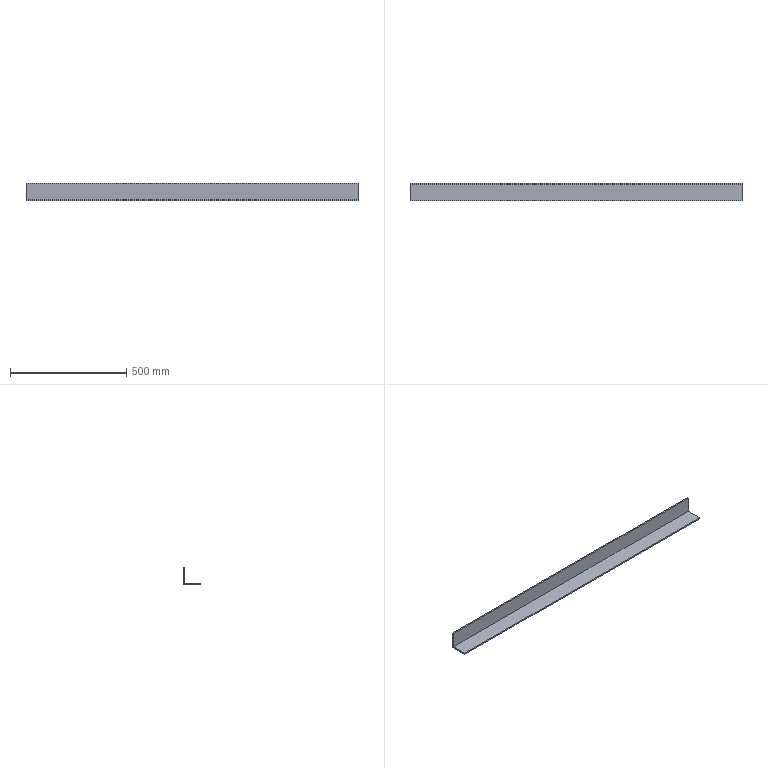Component | NX | DOWN_FRAME1430_2 | 1 solid | 8 faces | box 1430 x 75 x 75 mm | volume 1235520 mm3 | plane 8
STEP:
#1=CARTESIAN_POINT('',(0.,0.,0.));
#2=DIRECTION('',(0.,0.,1.));
#3=DIRECTION('',(1.,0.,0.));
#4=AXIS2_PLACEMENT_3D('',#1,#2,#3);
#5=CARTESIAN_POINT('',(0.,-6.,75.));
#6=VERTEX_POINT('',#5);
#7=CARTESIAN_POINT('',(0.,-6.,6.));
#8=VERTEX_POINT('',#7);
#9=CARTESIAN_POINT('',(0.,-6.,75.));
#10=DIRECTION('',(0.,0.,-1.));
#11=VECTOR('',#10,1.);
#12=LINE('',#9,#11);
#13=CARTESIAN_POINT('',(1430.,-6.,75.));
#14=DIRECTION('',(0.,1.,0.));
#15=DIRECTION('',(-1.,0.,0.));
#16=AXIS2_PLACEMENT_3D('',#13,#14,#15);
#17=PLANE('',#16);
#18=CARTESIAN_POINT('',(1430.,0.));
#19=DIRECTION('',(0.,-1.));
#20=VECTOR('',#19,1.);
#21=LINE('',#18,#20);
#22=(GEOMETRIC_REPRESENTATION_CONTEXT(2)PARAMETRIC_REPRESENTATION_CONTEXT()REPRESENTATION_CONTEXT('',''));
#23=DEFINITIONAL_REPRESENTATION('',(#21),#22);
#24=PCURVE('',#17,#23);
#25=CARTESIAN_POINT('',(0.,-6.,6.));
#26=DIRECTION('',(-1.,0.,0.));
#27=DIRECTION('',(0.,-1.,0.));
#28=AXIS2_PLACEMENT_3D('',#25,#26,#27);
#29=PLANE('',#28);
#30=CARTESIAN_POINT('',(0.,69.));
#31=DIRECTION('',(0.,-1.));
#32=VECTOR('',#31,1.);
#33=LINE('',#30,#32);
#34=(GEOMETRIC_REPRESENTATION_CONTEXT(2)PARAMETRIC_REPRESENTATION_CONTEXT()REPRESENTATION_CONTEXT('',''));
#35=DEFINITIONAL_REPRESENTATION('',(#33),#34);
#36=PCURVE('',#29,#35);
#37=SURFACE_CURVE('',#12,(#24,#36),.PCURVE_S1.);
#38=EDGE_CURVE('',#6,#8,#37,.T.);
#39=ORIENTED_EDGE('',*,*,#38,.T.);
#40=CARTESIAN_POINT('',(1430.,-6.,6.));
#41=VERTEX_POINT('',#40);
#42=CARTESIAN_POINT('',(1430.,-6.,6.));
#43=DIRECTION('',(-1.,0.,0.));
#44=VECTOR('',#43,1.);
#45=LINE('',#42,#44);
#46=CARTESIAN_POINT('',(0.,-69.));
#47=DIRECTION('',(1.,0.));
#48=VECTOR('',#47,1.);
#49=LINE('',#46,#48);
#50=(GEOMETRIC_REPRESENTATION_CONTEXT(2)PARAMETRIC_REPRESENTATION_CONTEXT()REPRESENTATION_CONTEXT('',''));
#51=DEFINITIONAL_REPRESENTATION('',(#49),#50);
#52=PCURVE('',#17,#51);
#53=CARTESIAN_POINT('',(1430.,-6.,6.));
#54=DIRECTION('',(0.,-0.,-1.));
#55=DIRECTION('',(0.,1.,-0.));
#56=AXIS2_PLACEMENT_3D('',#53,#54,#55);
#57=PLANE('',#56);
#58=CARTESIAN_POINT('',(0.,0.));
#59=DIRECTION('',(0.,-1.));
#60=VECTOR('',#59,1.);
#61=LINE('',#58,#60);
#62=(GEOMETRIC_REPRESENTATION_CONTEXT(2)PARAMETRIC_REPRESENTATION_CONTEXT()REPRESENTATION_CONTEXT('',''));
#63=DEFINITIONAL_REPRESENTATION('',(#61),#62);
#64=PCURVE('',#57,#63);
#65=SURFACE_CURVE('',#45,(#52,#64),.PCURVE_S1.);
#66=EDGE_CURVE('',#41,#8,#65,.T.);
#67=ORIENTED_EDGE('',*,*,#66,.F.);
#68=CARTESIAN_POINT('',(1430.,-6.,75.));
#69=VERTEX_POINT('',#68);
#70=CARTESIAN_POINT('',(1430.,-6.,75.));
#71=DIRECTION('',(0.,0.,-1.));
#72=VECTOR('',#71,1.);
#73=LINE('',#70,#72);
#74=CARTESIAN_POINT('',(0.,0.));
#75=DIRECTION('',(0.,-1.));
#76=VECTOR('',#75,1.);
#77=LINE('',#74,#76);
#78=(GEOMETRIC_REPRESENTATION_CONTEXT(2)PARAMETRIC_REPRESENTATION_CONTEXT()REPRESENTATION_CONTEXT('',''));
#79=DEFINITIONAL_REPRESENTATION('',(#77),#78);
#80=PCURVE('',#17,#79);
#81=CARTESIAN_POINT('',(1430.,-6.,6.));
#82=DIRECTION('',(-1.,0.,0.));
#83=DIRECTION('',(0.,-1.,0.));
#84=AXIS2_PLACEMENT_3D('',#81,#82,#83);
#85=PLANE('',#84);
#86=CARTESIAN_POINT('',(0.,69.));
#87=DIRECTION('',(0.,-1.));
#88=VECTOR('',#87,1.);
#89=LINE('',#86,#88);
#90=(GEOMETRIC_REPRESENTATION_CONTEXT(2)PARAMETRIC_REPRESENTATION_CONTEXT()REPRESENTATION_CONTEXT('',''));
#91=DEFINITIONAL_REPRESENTATION('',(#89),#90);
#92=PCURVE('',#85,#91);
#93=SURFACE_CURVE('',#73,(#80,#92),.PCURVE_S1.);
#94=EDGE_CURVE('',#69,#41,#93,.T.);
#95=ORIENTED_EDGE('',*,*,#94,.F.);
#96=CARTESIAN_POINT('',(1430.,-6.,75.));
#97=DIRECTION('',(-1.,0.,0.));
#98=VECTOR('',#97,1.);
#99=LINE('',#96,#98);
#100=CARTESIAN_POINT('',(0.,0.));
#101=DIRECTION('',(1.,0.));
#102=VECTOR('',#101,1.);
#103=LINE('',#100,#102);
#104=(GEOMETRIC_REPRESENTATION_CONTEXT(2)PARAMETRIC_REPRESENTATION_CONTEXT()REPRESENTATION_CONTEXT('',''));
#105=DEFINITIONAL_REPRESENTATION('',(#103),#104);
#106=PCURVE('',#17,#105);
#107=CARTESIAN_POINT('',(1430.,0.,75.));
#108=DIRECTION('',(0.,0.,-1.));
#109=DIRECTION('',(0.,1.,0.));
#110=AXIS2_PLACEMENT_3D('',#107,#108,#109);
#111=PLANE('',#110);
#112=CARTESIAN_POINT('',(-6.,0.));
#113=DIRECTION('',(0.,-1.));
#114=VECTOR('',#113,1.);
#115=LINE('',#112,#114);
#116=(GEOMETRIC_REPRESENTATION_CONTEXT(2)PARAMETRIC_REPRESENTATION_CONTEXT()REPRESENTATION_CONTEXT('',''));
#117=DEFINITIONAL_REPRESENTATION('',(#115),#116);
#118=PCURVE('',#111,#117);
#119=SURFACE_CURVE('',#99,(#106,#118),.PCURVE_S1.);
#120=EDGE_CURVE('',#69,#6,#119,.T.);
#121=ORIENTED_EDGE('',*,*,#120,.T.);
#122=EDGE_LOOP('',(#39,#67,#95,#121));
#123=FACE_BOUND('',#122,.T.);
#124=ADVANCED_FACE('',(#123),#17,.F.);
#125=CARTESIAN_POINT('',(0.,-75.,6.));
#126=VERTEX_POINT('',#125);
#127=CARTESIAN_POINT('',(0.,-6.,6.));
#128=DIRECTION('',(0.,-1.,0.));
#129=VECTOR('',#128,1.);
#130=LINE('',#127,#129);
#131=CARTESIAN_POINT('',(0.,-1430.));
#132=DIRECTION('',(-1.,0.));
#133=VECTOR('',#132,1.);
#134=LINE('',#131,#133);
#135=(GEOMETRIC_REPRESENTATION_CONTEXT(2)PARAMETRIC_REPRESENTATION_CONTEXT()REPRESENTATION_CONTEXT('',''));
#136=DEFINITIONAL_REPRESENTATION('',(#134),#135);
#137=PCURVE('',#57,#136);
#138=CARTESIAN_POINT('',(0.,0.));
#139=DIRECTION('',(1.,0.));
#140=VECTOR('',#139,1.);
#141=LINE('',#138,#140);
#142=(GEOMETRIC_REPRESENTATION_CONTEXT(2)PARAMETRIC_REPRESENTATION_CONTEXT()REPRESENTATION_CONTEXT('',''));
#143=DEFINITIONAL_REPRESENTATION('',(#141),#142);
#144=PCURVE('',#29,#143);
#145=SURFACE_CURVE('',#130,(#137,#144),.PCURVE_S1.);
#146=EDGE_CURVE('',#8,#126,#145,.T.);
#147=ORIENTED_EDGE('',*,*,#146,.T.);
#148=CARTESIAN_POINT('',(1430.,-75.,6.));
#149=VERTEX_POINT('',#148);
#150=CARTESIAN_POINT('',(1430.,-75.,6.));
#151=DIRECTION('',(-1.,0.,0.));
#152=VECTOR('',#151,1.);
#153=LINE('',#150,#152);
#154=CARTESIAN_POINT('',(-69.,0.));
#155=DIRECTION('',(0.,-1.));
#156=VECTOR('',#155,1.);
#157=LINE('',#154,#156);
#158=(GEOMETRIC_REPRESENTATION_CONTEXT(2)PARAMETRIC_REPRESENTATION_CONTEXT()REPRESENTATION_CONTEXT('',''));
#159=DEFINITIONAL_REPRESENTATION('',(#157),#158);
#160=PCURVE('',#57,#159);
#161=CARTESIAN_POINT('',(1430.,-75.,6.));
#162=DIRECTION('',(0.,1.,0.));
#163=DIRECTION('',(-1.,0.,0.));
#164=AXIS2_PLACEMENT_3D('',#161,#162,#163);
#165=PLANE('',#164);
#166=CARTESIAN_POINT('',(0.,0.));
#167=DIRECTION('',(1.,0.));
#168=VECTOR('',#167,1.);
#169=LINE('',#166,#168);
#170=(GEOMETRIC_REPRESENTATION_CONTEXT(2)PARAMETRIC_REPRESENTATION_CONTEXT()REPRESENTATION_CONTEXT('',''));
#171=DEFINITIONAL_REPRESENTATION('',(#169),#170);
#172=PCURVE('',#165,#171);
#173=SURFACE_CURVE('',#153,(#160,#172),.PCURVE_S1.);
#174=EDGE_CURVE('',#149,#126,#173,.T.);
#175=ORIENTED_EDGE('',*,*,#174,.F.);
#176=CARTESIAN_POINT('',(1430.,-6.,6.));
#177=DIRECTION('',(0.,-1.,0.));
#178=VECTOR('',#177,1.);
#179=LINE('',#176,#178);
#180=CARTESIAN_POINT('',(0.,0.));
#181=DIRECTION('',(-1.,0.));
#182=VECTOR('',#181,1.);
#183=LINE('',#180,#182);
#184=(GEOMETRIC_REPRESENTATION_CONTEXT(2)PARAMETRIC_REPRESENTATION_CONTEXT()REPRESENTATION_CONTEXT('',''));
#185=DEFINITIONAL_REPRESENTATION('',(#183),#184);
#186=PCURVE('',#57,#185);
#187=CARTESIAN_POINT('',(0.,0.));
#188=DIRECTION('',(1.,0.));
#189=VECTOR('',#188,1.);
#190=LINE('',#187,#189);
#191=(GEOMETRIC_REPRESENTATION_CONTEXT(2)PARAMETRIC_REPRESENTATION_CONTEXT()REPRESENTATION_CONTEXT('',''));
#192=DEFINITIONAL_REPRESENTATION('',(#190),#191);
#193=PCURVE('',#85,#192);
#194=SURFACE_CURVE('',#179,(#186,#193),.PCURVE_S1.);
#195=EDGE_CURVE('',#41,#149,#194,.T.);
#196=ORIENTED_EDGE('',*,*,#195,.F.);
#197=ORIENTED_EDGE('',*,*,#66,.T.);
#198=EDGE_LOOP('',(#147,#175,#196,#197));
#199=FACE_BOUND('',#198,.T.);
#200=ADVANCED_FACE('',(#199),#57,.F.);
#201=CARTESIAN_POINT('',(0.,-75.,0.));
#202=VERTEX_POINT('',#201);
#203=CARTESIAN_POINT('',(0.,-75.,6.));
#204=DIRECTION('',(0.,0.,-1.));
#205=VECTOR('',#204,1.);
#206=LINE('',#203,#205);
#207=CARTESIAN_POINT('',(1430.,0.));
#208=DIRECTION('',(0.,-1.));
#209=VECTOR('',#208,1.);
#210=LINE('',#207,#209);
#211=(GEOMETRIC_REPRESENTATION_CONTEXT(2)PARAMETRIC_REPRESENTATION_CONTEXT()REPRESENTATION_CONTEXT('',''));
#212=DEFINITIONAL_REPRESENTATION('',(#210),#211);
#213=PCURVE('',#165,#212);
#214=CARTESIAN_POINT('',(69.,0.));
#215=DIRECTION('',(0.,-1.));
#216=VECTOR('',#215,1.);
#217=LINE('',#214,#216);
#218=(GEOMETRIC_REPRESENTATION_CONTEXT(2)PARAMETRIC_REPRESENTATION_CONTEXT()REPRESENTATION_CONTEXT('',''));
#219=DEFINITIONAL_REPRESENTATION('',(#217),#218);
#220=PCURVE('',#29,#219);
#221=SURFACE_CURVE('',#206,(#213,#220),.PCURVE_S1.);
#222=EDGE_CURVE('',#126,#202,#221,.T.);
#223=ORIENTED_EDGE('',*,*,#222,.T.);
#224=CARTESIAN_POINT('',(1430.,-75.,0.));
#225=VERTEX_POINT('',#224);
#226=CARTESIAN_POINT('',(1430.,-75.,0.));
#227=DIRECTION('',(-1.,0.,0.));
#228=VECTOR('',#227,1.);
#229=LINE('',#226,#228);
#230=CARTESIAN_POINT('',(0.,-6.));
#231=DIRECTION('',(1.,0.));
#232=VECTOR('',#231,1.);
#233=LINE('',#230,#232);
#234=(GEOMETRIC_REPRESENTATION_CONTEXT(2)PARAMETRIC_REPRESENTATION_CONTEXT()REPRESENTATION_CONTEXT('',''));
#235=DEFINITIONAL_REPRESENTATION('',(#233),#234);
#236=PCURVE('',#165,#235);
#237=CARTESIAN_POINT('',(1430.,-75.,0.));
#238=DIRECTION('',(0.,0.,1.));
#239=DIRECTION('',(0.,-1.,0.));
#240=AXIS2_PLACEMENT_3D('',#237,#238,#239);
#241=PLANE('',#240);
#242=CARTESIAN_POINT('',(0.,0.));
#243=DIRECTION('',(0.,-1.));
#244=VECTOR('',#243,1.);
#245=LINE('',#242,#244);
#246=(GEOMETRIC_REPRESENTATION_CONTEXT(2)PARAMETRIC_REPRESENTATION_CONTEXT()REPRESENTATION_CONTEXT('',''));
#247=DEFINITIONAL_REPRESENTATION('',(#245),#246);
#248=PCURVE('',#241,#247);
#249=SURFACE_CURVE('',#229,(#236,#248),.PCURVE_S1.);
#250=EDGE_CURVE('',#225,#202,#249,.T.);
#251=ORIENTED_EDGE('',*,*,#250,.F.);
#252=CARTESIAN_POINT('',(1430.,-75.,6.));
#253=DIRECTION('',(0.,0.,-1.));
#254=VECTOR('',#253,1.);
#255=LINE('',#252,#254);
#256=CARTESIAN_POINT('',(0.,0.));
#257=DIRECTION('',(0.,-1.));
#258=VECTOR('',#257,1.);
#259=LINE('',#256,#258);
#260=(GEOMETRIC_REPRESENTATION_CONTEXT(2)PARAMETRIC_REPRESENTATION_CONTEXT()REPRESENTATION_CONTEXT('',''));
#261=DEFINITIONAL_REPRESENTATION('',(#259),#260);
#262=PCURVE('',#165,#261);
#263=CARTESIAN_POINT('',(69.,0.));
#264=DIRECTION('',(0.,-1.));
#265=VECTOR('',#264,1.);
#266=LINE('',#263,#265);
#267=(GEOMETRIC_REPRESENTATION_CONTEXT(2)PARAMETRIC_REPRESENTATION_CONTEXT()REPRESENTATION_CONTEXT('',''));
#268=DEFINITIONAL_REPRESENTATION('',(#266),#267);
#269=PCURVE('',#85,#268);
#270=SURFACE_CURVE('',#255,(#262,#269),.PCURVE_S1.);
#271=EDGE_CURVE('',#149,#225,#270,.T.);
#272=ORIENTED_EDGE('',*,*,#271,.F.);
#273=ORIENTED_EDGE('',*,*,#174,.T.);
#274=EDGE_LOOP('',(#223,#251,#272,#273));
#275=FACE_BOUND('',#274,.T.);
#276=ADVANCED_FACE('',(#275),#165,.F.);
#277=CARTESIAN_POINT('',(0.,0.,0.));
#278=VERTEX_POINT('',#277);
#279=CARTESIAN_POINT('',(0.,-75.,0.));
#280=DIRECTION('',(0.,1.,-0.));
#281=VECTOR('',#280,1.);
#282=LINE('',#279,#281);
#283=CARTESIAN_POINT('',(0.,-1430.));
#284=DIRECTION('',(-1.,0.));
#285=VECTOR('',#284,1.);
#286=LINE('',#283,#285);
#287=(GEOMETRIC_REPRESENTATION_CONTEXT(2)PARAMETRIC_REPRESENTATION_CONTEXT()REPRESENTATION_CONTEXT('',''));
#288=DEFINITIONAL_REPRESENTATION('',(#286),#287);
#289=PCURVE('',#241,#288);
#290=CARTESIAN_POINT('',(69.,-6.));
#291=DIRECTION('',(-1.,-0.));
#292=VECTOR('',#291,1.);
#293=LINE('',#290,#292);
#294=(GEOMETRIC_REPRESENTATION_CONTEXT(2)PARAMETRIC_REPRESENTATION_CONTEXT()REPRESENTATION_CONTEXT('',''));
#295=DEFINITIONAL_REPRESENTATION('',(#293),#294);
#296=PCURVE('',#29,#295);
#297=SURFACE_CURVE('',#282,(#289,#296),.PCURVE_S1.);
#298=EDGE_CURVE('',#202,#278,#297,.T.);
#299=ORIENTED_EDGE('',*,*,#298,.T.);
#300=CARTESIAN_POINT('',(1430.,0.,0.));
#301=VERTEX_POINT('',#300);
#302=CARTESIAN_POINT('',(1430.,0.,0.));
#303=DIRECTION('',(-1.,0.,0.));
#304=VECTOR('',#303,1.);
#305=LINE('',#302,#304);
#306=CARTESIAN_POINT('',(-75.,0.));
#307=DIRECTION('',(0.,-1.));
#308=VECTOR('',#307,1.);
#309=LINE('',#306,#308);
#310=(GEOMETRIC_REPRESENTATION_CONTEXT(2)PARAMETRIC_REPRESENTATION_CONTEXT()REPRESENTATION_CONTEXT('',''));
#311=DEFINITIONAL_REPRESENTATION('',(#309),#310);
#312=PCURVE('',#241,#311);
#313=CARTESIAN_POINT('',(1430.,0.,0.));
#314=DIRECTION('',(0.,-1.,0.));
#315=DIRECTION('',(1.,0.,0.));
#316=AXIS2_PLACEMENT_3D('',#313,#314,#315);
#317=PLANE('',#316);
#318=CARTESIAN_POINT('',(0.,0.));
#319=DIRECTION('',(-1.,0.));
#320=VECTOR('',#319,1.);
#321=LINE('',#318,#320);
#322=(GEOMETRIC_REPRESENTATION_CONTEXT(2)PARAMETRIC_REPRESENTATION_CONTEXT()REPRESENTATION_CONTEXT('',''));
#323=DEFINITIONAL_REPRESENTATION('',(#321),#322);
#324=PCURVE('',#317,#323);
#325=SURFACE_CURVE('',#305,(#312,#324),.PCURVE_S1.);
#326=EDGE_CURVE('',#301,#278,#325,.T.);
#327=ORIENTED_EDGE('',*,*,#326,.F.);
#328=CARTESIAN_POINT('',(1430.,-75.,0.));
#329=DIRECTION('',(0.,1.,-0.));
#330=VECTOR('',#329,1.);
#331=LINE('',#328,#330);
#332=CARTESIAN_POINT('',(0.,0.));
#333=DIRECTION('',(-1.,0.));
#334=VECTOR('',#333,1.);
#335=LINE('',#332,#334);
#336=(GEOMETRIC_REPRESENTATION_CONTEXT(2)PARAMETRIC_REPRESENTATION_CONTEXT()REPRESENTATION_CONTEXT('',''));
#337=DEFINITIONAL_REPRESENTATION('',(#335),#336);
#338=PCURVE('',#241,#337);
#339=CARTESIAN_POINT('',(69.,-6.));
#340=DIRECTION('',(-1.,-0.));
#341=VECTOR('',#340,1.);
#342=LINE('',#339,#341);
#343=(GEOMETRIC_REPRESENTATION_CONTEXT(2)PARAMETRIC_REPRESENTATION_CONTEXT()REPRESENTATION_CONTEXT('',''));
#344=DEFINITIONAL_REPRESENTATION('',(#342),#343);
#345=PCURVE('',#85,#344);
#346=SURFACE_CURVE('',#331,(#338,#345),.PCURVE_S1.);
#347=EDGE_CURVE('',#225,#301,#346,.T.);
#348=ORIENTED_EDGE('',*,*,#347,.F.);
#349=ORIENTED_EDGE('',*,*,#250,.T.);
#350=EDGE_LOOP('',(#299,#327,#348,#349));
#351=FACE_BOUND('',#350,.T.);
#352=ADVANCED_FACE('',(#351),#241,.F.);
#353=CARTESIAN_POINT('',(0.,0.,75.));
#354=VERTEX_POINT('',#353);
#355=CARTESIAN_POINT('',(0.,0.,0.));
#356=DIRECTION('',(0.,0.,1.));
#357=VECTOR('',#356,1.);
#358=LINE('',#355,#357);
#359=CARTESIAN_POINT('',(-1430.,0.));
#360=DIRECTION('',(0.,1.));
#361=VECTOR('',#360,1.);
#362=LINE('',#359,#361);
#363=(GEOMETRIC_REPRESENTATION_CONTEXT(2)PARAMETRIC_REPRESENTATION_CONTEXT()REPRESENTATION_CONTEXT('',''));
#364=DEFINITIONAL_REPRESENTATION('',(#362),#363);
#365=PCURVE('',#317,#364);
#366=CARTESIAN_POINT('',(-6.,-6.));
#367=DIRECTION('',(0.,1.));
#368=VECTOR('',#367,1.);
#369=LINE('',#366,#368);
#370=(GEOMETRIC_REPRESENTATION_CONTEXT(2)PARAMETRIC_REPRESENTATION_CONTEXT()REPRESENTATION_CONTEXT('',''));
#371=DEFINITIONAL_REPRESENTATION('',(#369),#370);
#372=PCURVE('',#29,#371);
#373=SURFACE_CURVE('',#358,(#365,#372),.PCURVE_S1.);
#374=EDGE_CURVE('',#278,#354,#373,.T.);
#375=ORIENTED_EDGE('',*,*,#374,.T.);
#376=CARTESIAN_POINT('',(1430.,0.,75.));
#377=VERTEX_POINT('',#376);
#378=CARTESIAN_POINT('',(1430.,0.,75.));
#379=DIRECTION('',(-1.,0.,0.));
#380=VECTOR('',#379,1.);
#381=LINE('',#378,#380);
#382=CARTESIAN_POINT('',(0.,75.));
#383=DIRECTION('',(-1.,0.));
#384=VECTOR('',#383,1.);
#385=LINE('',#382,#384);
#386=(GEOMETRIC_REPRESENTATION_CONTEXT(2)PARAMETRIC_REPRESENTATION_CONTEXT()REPRESENTATION_CONTEXT('',''));
#387=DEFINITIONAL_REPRESENTATION('',(#385),#386);
#388=PCURVE('',#317,#387);
#389=CARTESIAN_POINT('',(0.,0.));
#390=DIRECTION('',(0.,-1.));
#391=VECTOR('',#390,1.);
#392=LINE('',#389,#391);
#393=(GEOMETRIC_REPRESENTATION_CONTEXT(2)PARAMETRIC_REPRESENTATION_CONTEXT()REPRESENTATION_CONTEXT('',''));
#394=DEFINITIONAL_REPRESENTATION('',(#392),#393);
#395=PCURVE('',#111,#394);
#396=SURFACE_CURVE('',#381,(#388,#395),.PCURVE_S1.);
#397=EDGE_CURVE('',#377,#354,#396,.T.);
#398=ORIENTED_EDGE('',*,*,#397,.F.);
#399=CARTESIAN_POINT('',(1430.,0.,0.));
#400=DIRECTION('',(0.,0.,1.));
#401=VECTOR('',#400,1.);
#402=LINE('',#399,#401);
#403=CARTESIAN_POINT('',(0.,0.));
#404=DIRECTION('',(0.,1.));
#405=VECTOR('',#404,1.);
#406=LINE('',#403,#405);
#407=(GEOMETRIC_REPRESENTATION_CONTEXT(2)PARAMETRIC_REPRESENTATION_CONTEXT()REPRESENTATION_CONTEXT('',''));
#408=DEFINITIONAL_REPRESENTATION('',(#406),#407);
#409=PCURVE('',#317,#408);
#410=CARTESIAN_POINT('',(-6.,-6.));
#411=DIRECTION('',(0.,1.));
#412=VECTOR('',#411,1.);
#413=LINE('',#410,#412);
#414=(GEOMETRIC_REPRESENTATION_CONTEXT(2)PARAMETRIC_REPRESENTATION_CONTEXT()REPRESENTATION_CONTEXT('',''));
#415=DEFINITIONAL_REPRESENTATION('',(#413),#414);
#416=PCURVE('',#85,#415);
#417=SURFACE_CURVE('',#402,(#409,#416),.PCURVE_S1.);
#418=EDGE_CURVE('',#301,#377,#417,.T.);
#419=ORIENTED_EDGE('',*,*,#418,.F.);
#420=ORIENTED_EDGE('',*,*,#326,.T.);
#421=EDGE_LOOP('',(#375,#398,#419,#420));
#422=FACE_BOUND('',#421,.T.);
#423=ADVANCED_FACE('',(#422),#317,.F.);
#424=CARTESIAN_POINT('',(0.,0.,75.));
#425=DIRECTION('',(0.,-1.,0.));
#426=VECTOR('',#425,1.);
#427=LINE('',#424,#426);
#428=CARTESIAN_POINT('',(0.,-1430.));
#429=DIRECTION('',(-1.,0.));
#430=VECTOR('',#429,1.);
#431=LINE('',#428,#430);
#432=(GEOMETRIC_REPRESENTATION_CONTEXT(2)PARAMETRIC_REPRESENTATION_CONTEXT()REPRESENTATION_CONTEXT('',''));
#433=DEFINITIONAL_REPRESENTATION('',(#431),#432);
#434=PCURVE('',#111,#433);
#435=CARTESIAN_POINT('',(-6.,69.));
#436=DIRECTION('',(1.,0.));
#437=VECTOR('',#436,1.);
#438=LINE('',#435,#437);
#439=(GEOMETRIC_REPRESENTATION_CONTEXT(2)PARAMETRIC_REPRESENTATION_CONTEXT()REPRESENTATION_CONTEXT('',''));
#440=DEFINITIONAL_REPRESENTATION('',(#438),#439);
#441=PCURVE('',#29,#440);
#442=SURFACE_CURVE('',#427,(#434,#441),.PCURVE_S1.);
#443=EDGE_CURVE('',#354,#6,#442,.T.);
#444=ORIENTED_EDGE('',*,*,#443,.T.);
#445=ORIENTED_EDGE('',*,*,#120,.F.);
#446=CARTESIAN_POINT('',(1430.,0.,75.));
#447=DIRECTION('',(0.,-1.,0.));
#448=VECTOR('',#447,1.);
#449=LINE('',#446,#448);
#450=CARTESIAN_POINT('',(0.,0.));
#451=DIRECTION('',(-1.,0.));
#452=VECTOR('',#451,1.);
#453=LINE('',#450,#452);
#454=(GEOMETRIC_REPRESENTATION_CONTEXT(2)PARAMETRIC_REPRESENTATION_CONTEXT()REPRESENTATION_CONTEXT('',''));
#455=DEFINITIONAL_REPRESENTATION('',(#453),#454);
#456=PCURVE('',#111,#455);
#457=CARTESIAN_POINT('',(-6.,69.));
#458=DIRECTION('',(1.,0.));
#459=VECTOR('',#458,1.);
#460=LINE('',#457,#459);
#461=(GEOMETRIC_REPRESENTATION_CONTEXT(2)PARAMETRIC_REPRESENTATION_CONTEXT()REPRESENTATION_CONTEXT('',''));
#462=DEFINITIONAL_REPRESENTATION('',(#460),#461);
#463=PCURVE('',#85,#462);
#464=SURFACE_CURVE('',#449,(#456,#463),.PCURVE_S1.);
#465=EDGE_CURVE('',#377,#69,#464,.T.);
#466=ORIENTED_EDGE('',*,*,#465,.F.);
#467=ORIENTED_EDGE('',*,*,#397,.T.);
#468=EDGE_LOOP('',(#444,#445,#466,#467));
#469=FACE_BOUND('',#468,.T.);
#470=ADVANCED_FACE('',(#469),#111,.F.);
#471=ORIENTED_EDGE('',*,*,#94,.T.);
#472=ORIENTED_EDGE('',*,*,#195,.T.);
#473=ORIENTED_EDGE('',*,*,#271,.T.);
#474=ORIENTED_EDGE('',*,*,#347,.T.);
#475=ORIENTED_EDGE('',*,*,#418,.T.);
#476=ORIENTED_EDGE('',*,*,#465,.T.);
#477=EDGE_LOOP('',(#471,#472,#473,#474,#475,#476));
#478=FACE_BOUND('',#477,.T.);
#479=ADVANCED_FACE('',(#478),#85,.F.);
#480=ORIENTED_EDGE('',*,*,#38,.F.);
#481=ORIENTED_EDGE('',*,*,#443,.F.);
#482=ORIENTED_EDGE('',*,*,#374,.F.);
#483=ORIENTED_EDGE('',*,*,#298,.F.);
#484=ORIENTED_EDGE('',*,*,#222,.F.);
#485=ORIENTED_EDGE('',*,*,#146,.F.);
#486=EDGE_LOOP('',(#480,#481,#482,#483,#484,#485));
#487=FACE_BOUND('',#486,.T.);
#488=ADVANCED_FACE('',(#487),#29,.T.);
#489=CLOSED_SHELL('',(#124,#200,#276,#352,#423,#470,#479,#488));
#490=MANIFOLD_SOLID_BREP('',#489);
#491=(LENGTH_UNIT()NAMED_UNIT(*)SI_UNIT(.MILLI.,.METRE.));
#492=UNCERTAINTY_MEASURE_WITH_UNIT(LENGTH_MEASURE(0.0000001),#491,'','');
#493=(NAMED_UNIT(*)PLANE_ANGLE_UNIT()SI_UNIT($,.RADIAN.));
#494=(NAMED_UNIT(*)SI_UNIT($,.STERADIAN.)SOLID_ANGLE_UNIT());
#495=(GEOMETRIC_REPRESENTATION_CONTEXT(3)GLOBAL_UNCERTAINTY_ASSIGNED_CONTEXT((#492))GLOBAL_UNIT_ASSIGNED_CONTEXT((#491,#493,#494))REPRESENTATION_CONTEXT('',''));
#496=ADVANCED_BREP_SHAPE_REPRESENTATION('',(#4,#490),#495);